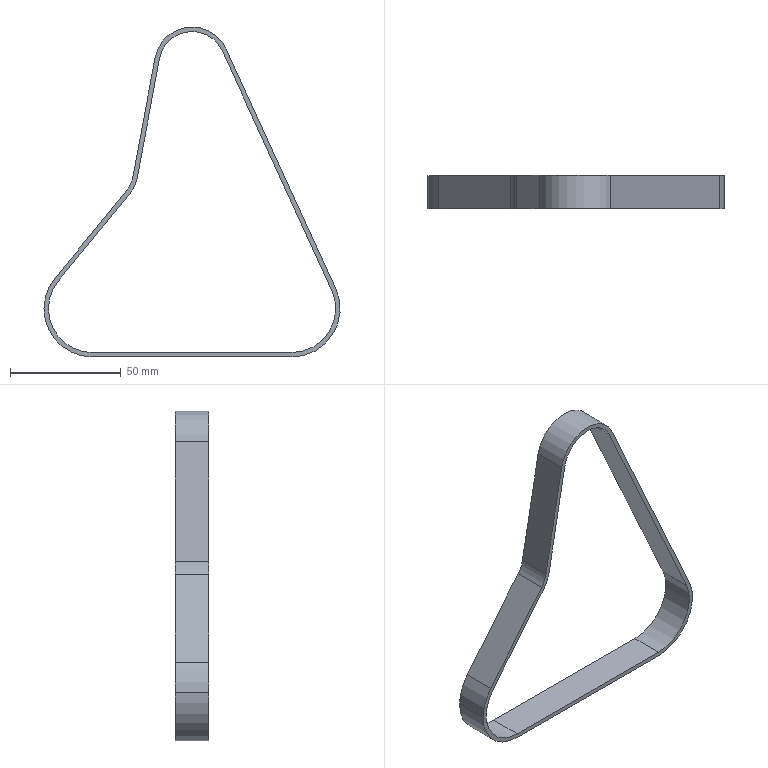Component | SolidWorks | Belt11-1 | 1 solid | 20 faces | box 133.44 x 15 x 148.67 mm | volume 13508 mm3 | cylinder 10 | plane 10 | commonest cylinder face diameters 39.44 x3 43.44 x3 33.89 x1 29.89 x1 26 x1 30 x1
STEP:
#1=COLOUR_RGB('',0.7922,0.8196,0.9333);
#2=FILL_AREA_STYLE_COLOUR('',#1);
#3=FILL_AREA_STYLE('',(#2));
#4=SURFACE_STYLE_FILL_AREA(#3);
#5=SURFACE_SIDE_STYLE('',(#4));
#6=SURFACE_STYLE_USAGE(.BOTH.,#5);
#7=PRESENTATION_STYLE_ASSIGNMENT((#6));
#8=CARTESIAN_POINT('',(-0.317,-0.7841,16.584));
#9=VERTEX_POINT('',#8);
#10=CARTESIAN_POINT('',(-0.4928,-0.7841,16.092));
#11=VERTEX_POINT('',#10);
#12=CARTESIAN_POINT('',(0.2836,-0.7841,16.092));
#13=DIRECTION('',(0.,-1.,0.));
#14=DIRECTION('',(1.,0.,0.));
#15=AXIS2_PLACEMENT_3D('',#12,#13,#14);
#16=CIRCLE('',#15,0.7764);
#17=EDGE_CURVE('',#9,#11,#16,.T.);
#18=ORIENTED_EDGE('',*,*,#17,.T.);
#19=CARTESIAN_POINT('',(-0.4928,-0.1935,16.092));
#20=VERTEX_POINT('',#19);
#21=CARTESIAN_POINT('',(-0.4928,-0.7841,16.092));
#22=DIRECTION('',(0.,1.,0.));
#23=VECTOR('',#22,39.37);
#24=LINE('',#21,#23);
#25=EDGE_CURVE('',#11,#20,#24,.T.);
#26=ORIENTED_EDGE('',*,*,#25,.T.);
#27=CARTESIAN_POINT('',(-0.317,-0.1935,16.584));
#28=VERTEX_POINT('',#27);
#29=CARTESIAN_POINT('',(0.2836,-0.1935,16.092));
#30=DIRECTION('',(0.,-1.,0.));
#31=DIRECTION('',(1.,0.,0.));
#32=AXIS2_PLACEMENT_3D('',#29,#30,#31);
#33=CIRCLE('',#32,0.7764);
#34=EDGE_CURVE('',#28,#20,#33,.T.);
#35=ORIENTED_EDGE('',*,*,#34,.F.);
#36=CARTESIAN_POINT('',(-0.317,-0.7841,16.584));
#37=DIRECTION('',(0.,1.,0.));
#38=VECTOR('',#37,39.37);
#39=LINE('',#36,#38);
#40=EDGE_CURVE('',#9,#28,#39,.T.);
#41=ORIENTED_EDGE('',*,*,#40,.F.);
#42=EDGE_LOOP('',(#18,#26,#35,#41));
#43=FACE_OUTER_BOUND('',#42,.T.);
#44=CARTESIAN_POINT('',(0.2836,-0.7841,16.092));
#45=DIRECTION('',(0.,1.,0.));
#46=DIRECTION('',(-1.,0.,0.));
#47=AXIS2_PLACEMENT_3D('',#44,#45,#46);
#48=CYLINDRICAL_SURFACE('',#47,0.7764);
#49=ADVANCED_FACE('',(#43),#48,.F.);
#50=CARTESIAN_POINT('',(-0.5715,-0.7841,16.092));
#51=VERTEX_POINT('',#50);
#52=CARTESIAN_POINT('',(0.2836,-0.7841,15.237));
#53=VERTEX_POINT('',#52);
#54=CARTESIAN_POINT('',(0.2836,-0.7841,16.092));
#55=DIRECTION('',(0.,-1.,0.));
#56=DIRECTION('',(1.,0.,0.));
#57=AXIS2_PLACEMENT_3D('',#54,#55,#56);
#58=CIRCLE('',#57,0.8551);
#59=EDGE_CURVE('',#51,#53,#58,.T.);
#60=ORIENTED_EDGE('',*,*,#59,.F.);
#61=CARTESIAN_POINT('',(-0.5715,-0.1935,16.092));
#62=VERTEX_POINT('',#61);
#63=CARTESIAN_POINT('',(-0.5715,-0.7841,16.092));
#64=DIRECTION('',(0.,1.,0.));
#65=VECTOR('',#64,39.37);
#66=LINE('',#63,#65);
#67=EDGE_CURVE('',#51,#62,#66,.T.);
#68=ORIENTED_EDGE('',*,*,#67,.T.);
#69=CARTESIAN_POINT('',(0.2836,-0.1935,15.237));
#70=VERTEX_POINT('',#69);
#71=CARTESIAN_POINT('',(0.2836,-0.1935,16.092));
#72=DIRECTION('',(0.,-1.,0.));
#73=DIRECTION('',(1.,0.,0.));
#74=AXIS2_PLACEMENT_3D('',#71,#72,#73);
#75=CIRCLE('',#74,0.8551);
#76=EDGE_CURVE('',#62,#70,#75,.T.);
#77=ORIENTED_EDGE('',*,*,#76,.T.);
#78=CARTESIAN_POINT('',(0.2836,-0.7841,15.237));
#79=DIRECTION('',(0.,1.,0.));
#80=VECTOR('',#79,39.37);
#81=LINE('',#78,#80);
#82=EDGE_CURVE('',#53,#70,#81,.T.);
#83=ORIENTED_EDGE('',*,*,#82,.F.);
#84=EDGE_LOOP('',(#60,#68,#77,#83));
#85=FACE_OUTER_BOUND('',#84,.T.);
#86=CARTESIAN_POINT('',(0.2836,-0.7841,16.092));
#87=DIRECTION('',(0.,1.,0.));
#88=DIRECTION('',(-1.,0.,0.));
#89=AXIS2_PLACEMENT_3D('',#86,#87,#88);
#90=CYLINDRICAL_SURFACE('',#89,0.8551);
#91=ADVANCED_FACE('',(#85),#90,.T.);
#92=ORIENTED_EDGE('',*,*,#17,.F.);
#93=CARTESIAN_POINT('',(0.957,-0.7841,18.139));
#94=VERTEX_POINT('',#93);
#95=CARTESIAN_POINT('',(0.957,-0.7841,18.139));
#96=DIRECTION('',(0.6337,0.,0.7736));
#97=VECTOR('',#96,39.37);
#98=LINE('',#95,#97);
#99=EDGE_CURVE('',#9,#94,#98,.T.);
#100=ORIENTED_EDGE('',*,*,#99,.T.);
#101=CARTESIAN_POINT('',(1.081,-0.7841,18.405));
#102=VERTEX_POINT('',#101);
#103=CARTESIAN_POINT('',(0.5001,-0.7841,18.514));
#104=DIRECTION('',(0.,-1.,0.));
#105=DIRECTION('',(-1.,0.,0.));
#106=AXIS2_PLACEMENT_3D('',#103,#104,#105);
#107=CIRCLE('',#106,0.5906);
#108=EDGE_CURVE('',#94,#102,#107,.T.);
#109=ORIENTED_EDGE('',*,*,#108,.T.);
#110=CARTESIAN_POINT('',(1.477,-0.7841,20.531));
#111=VERTEX_POINT('',#110);
#112=CARTESIAN_POINT('',(1.477,-0.7841,20.531));
#113=DIRECTION('',(0.1832,0.,0.9831));
#114=VECTOR('',#113,39.37);
#115=LINE('',#112,#114);
#116=EDGE_CURVE('',#102,#111,#115,.T.);
#117=ORIENTED_EDGE('',*,*,#116,.T.);
#118=CARTESIAN_POINT('',(2.59,-0.7841,20.668));
#119=VERTEX_POINT('',#118);
#120=CARTESIAN_POINT('',(2.055,-0.7841,20.423));
#121=DIRECTION('',(0.,-1.,0.));
#122=DIRECTION('',(1.,0.,0.));
#123=AXIS2_PLACEMENT_3D('',#120,#121,#122);
#124=CIRCLE('',#123,0.5884);
#125=EDGE_CURVE('',#119,#111,#124,.T.);
#126=ORIENTED_EDGE('',*,*,#125,.F.);
#127=CARTESIAN_POINT('',(4.533,-0.7841,16.415));
#128=VERTEX_POINT('',#127);
#129=CARTESIAN_POINT('',(4.533,-0.7841,16.415));
#130=DIRECTION('',(-0.4155,0.,0.9096));
#131=VECTOR('',#130,39.37);
#132=LINE('',#129,#131);
#133=EDGE_CURVE('',#128,#119,#132,.T.);
#134=ORIENTED_EDGE('',*,*,#133,.F.);
#135=CARTESIAN_POINT('',(3.827,-0.7841,15.316));
#136=VERTEX_POINT('',#135);
#137=CARTESIAN_POINT('',(3.827,-0.7841,16.092));
#138=DIRECTION('',(0.,-1.,0.));
#139=DIRECTION('',(1.,0.,0.));
#140=AXIS2_PLACEMENT_3D('',#137,#138,#139);
#141=CIRCLE('',#140,0.7764);
#142=EDGE_CURVE('',#136,#128,#141,.T.);
#143=ORIENTED_EDGE('',*,*,#142,.F.);
#144=CARTESIAN_POINT('',(0.2836,-0.7841,15.316));
#145=VERTEX_POINT('',#144);
#146=CARTESIAN_POINT('',(0.2836,-0.7841,15.316));
#147=DIRECTION('',(1.,0.,-0.));
#148=VECTOR('',#147,39.37);
#149=LINE('',#146,#148);
#150=EDGE_CURVE('',#145,#136,#149,.T.);
#151=ORIENTED_EDGE('',*,*,#150,.F.);
#152=CARTESIAN_POINT('',(0.2836,-0.7841,16.092));
#153=DIRECTION('',(0.,-1.,0.));
#154=DIRECTION('',(1.,0.,0.));
#155=AXIS2_PLACEMENT_3D('',#152,#153,#154);
#156=CIRCLE('',#155,0.7764);
#157=EDGE_CURVE('',#11,#145,#156,.T.);
#158=ORIENTED_EDGE('',*,*,#157,.F.);
#159=EDGE_LOOP('',(#92,#100,#109,#117,#126,#134,#143,#151,#158));
#160=FACE_BOUND('',#159,.T.);
#161=CARTESIAN_POINT('',(0.896,-0.7841,18.189));
#162=VERTEX_POINT('',#161);
#163=CARTESIAN_POINT('',(-0.3779,-0.7841,16.634));
#164=VERTEX_POINT('',#163);
#165=CARTESIAN_POINT('',(-0.3779,-0.7841,16.634));
#166=DIRECTION('',(-0.6337,0.,-0.7736));
#167=VECTOR('',#166,39.37);
#168=LINE('',#165,#167);
#169=EDGE_CURVE('',#162,#164,#168,.T.);
#170=ORIENTED_EDGE('',*,*,#169,.T.);
#171=CARTESIAN_POINT('',(0.2836,-0.7841,16.092));
#172=DIRECTION('',(0.,-1.,0.));
#173=DIRECTION('',(1.,0.,0.));
#174=AXIS2_PLACEMENT_3D('',#171,#172,#173);
#175=CIRCLE('',#174,0.8551);
#176=EDGE_CURVE('',#164,#51,#175,.T.);
#177=ORIENTED_EDGE('',*,*,#176,.T.);
#178=ORIENTED_EDGE('',*,*,#59,.T.);
#179=CARTESIAN_POINT('',(3.827,-0.7841,15.237));
#180=VERTEX_POINT('',#179);
#181=CARTESIAN_POINT('',(0.2836,-0.7841,15.237));
#182=DIRECTION('',(1.,0.,-0.));
#183=VECTOR('',#182,39.37);
#184=LINE('',#181,#183);
#185=EDGE_CURVE('',#53,#180,#184,.T.);
#186=ORIENTED_EDGE('',*,*,#185,.T.);
#187=CARTESIAN_POINT('',(4.605,-0.7841,16.448));
#188=VERTEX_POINT('',#187);
#189=CARTESIAN_POINT('',(3.827,-0.7841,16.092));
#190=DIRECTION('',(0.,-1.,0.));
#191=DIRECTION('',(1.,0.,0.));
#192=AXIS2_PLACEMENT_3D('',#189,#190,#191);
#193=CIRCLE('',#192,0.8551);
#194=EDGE_CURVE('',#180,#188,#193,.T.);
#195=ORIENTED_EDGE('',*,*,#194,.T.);
#196=CARTESIAN_POINT('',(2.662,-0.7841,20.7));
#197=VERTEX_POINT('',#196);
#198=CARTESIAN_POINT('',(4.605,-0.7841,16.448));
#199=DIRECTION('',(-0.4155,0.,0.9096));
#200=VECTOR('',#199,39.37);
#201=LINE('',#198,#200);
#202=EDGE_CURVE('',#188,#197,#201,.T.);
#203=ORIENTED_EDGE('',*,*,#202,.T.);
#204=CARTESIAN_POINT('',(1.399,-0.7841,20.545));
#205=VERTEX_POINT('',#204);
#206=CARTESIAN_POINT('',(2.055,-0.7841,20.423));
#207=DIRECTION('',(0.,-1.,0.));
#208=DIRECTION('',(1.,0.,0.));
#209=AXIS2_PLACEMENT_3D('',#206,#207,#208);
#210=CIRCLE('',#209,0.6671);
#211=EDGE_CURVE('',#197,#205,#210,.T.);
#212=ORIENTED_EDGE('',*,*,#211,.T.);
#213=CARTESIAN_POINT('',(1.003,-0.7841,18.42));
#214=VERTEX_POINT('',#213);
#215=CARTESIAN_POINT('',(1.003,-0.7841,18.42));
#216=DIRECTION('',(-0.1832,0.,-0.9831));
#217=VECTOR('',#216,39.37);
#218=LINE('',#215,#217);
#219=EDGE_CURVE('',#205,#214,#218,.T.);
#220=ORIENTED_EDGE('',*,*,#219,.T.);
#221=CARTESIAN_POINT('',(0.5001,-0.7841,18.514));
#222=DIRECTION('',(0.,1.,0.));
#223=DIRECTION('',(1.,0.,0.));
#224=AXIS2_PLACEMENT_3D('',#221,#222,#223);
#225=CIRCLE('',#224,0.5118);
#226=EDGE_CURVE('',#214,#162,#225,.T.);
#227=ORIENTED_EDGE('',*,*,#226,.T.);
#228=EDGE_LOOP('',(#170,#177,#178,#186,#195,#203,#212,#220,#227));
#229=FACE_OUTER_BOUND('',#228,.T.);
#230=CARTESIAN_POINT('',(2.055,-0.7841,20.423));
#231=DIRECTION('',(0.,-1.,0.));
#232=DIRECTION('',(1.,0.,0.));
#233=AXIS2_PLACEMENT_3D('',#230,#231,#232);
#234=PLANE('',#233);
#235=ADVANCED_FACE('',(#160,#229),#234,.T.);
#236=CARTESIAN_POINT('',(0.957,-0.1935,18.139));
#237=VERTEX_POINT('',#236);
#238=CARTESIAN_POINT('',(0.957,-0.1935,18.139));
#239=DIRECTION('',(0.6337,0.,0.7736));
#240=VECTOR('',#239,39.37);
#241=LINE('',#238,#240);
#242=EDGE_CURVE('',#28,#237,#241,.T.);
#243=ORIENTED_EDGE('',*,*,#242,.F.);
#244=ORIENTED_EDGE('',*,*,#34,.T.);
#245=CARTESIAN_POINT('',(0.2836,-0.1935,15.316));
#246=VERTEX_POINT('',#245);
#247=CARTESIAN_POINT('',(0.2836,-0.1935,16.092));
#248=DIRECTION('',(0.,-1.,0.));
#249=DIRECTION('',(1.,0.,0.));
#250=AXIS2_PLACEMENT_3D('',#247,#248,#249);
#251=CIRCLE('',#250,0.7764);
#252=EDGE_CURVE('',#20,#246,#251,.T.);
#253=ORIENTED_EDGE('',*,*,#252,.T.);
#254=CARTESIAN_POINT('',(3.827,-0.1935,15.316));
#255=VERTEX_POINT('',#254);
#256=CARTESIAN_POINT('',(0.2836,-0.1935,15.316));
#257=DIRECTION('',(1.,0.,-0.));
#258=VECTOR('',#257,39.37);
#259=LINE('',#256,#258);
#260=EDGE_CURVE('',#246,#255,#259,.T.);
#261=ORIENTED_EDGE('',*,*,#260,.T.);
#262=CARTESIAN_POINT('',(4.533,-0.1935,16.415));
#263=VERTEX_POINT('',#262);
#264=CARTESIAN_POINT('',(3.827,-0.1935,16.092));
#265=DIRECTION('',(0.,-1.,0.));
#266=DIRECTION('',(1.,0.,0.));
#267=AXIS2_PLACEMENT_3D('',#264,#265,#266);
#268=CIRCLE('',#267,0.7764);
#269=EDGE_CURVE('',#255,#263,#268,.T.);
#270=ORIENTED_EDGE('',*,*,#269,.T.);
#271=CARTESIAN_POINT('',(2.59,-0.1935,20.668));
#272=VERTEX_POINT('',#271);
#273=CARTESIAN_POINT('',(4.533,-0.1935,16.415));
#274=DIRECTION('',(-0.4155,0.,0.9096));
#275=VECTOR('',#274,39.37);
#276=LINE('',#273,#275);
#277=EDGE_CURVE('',#263,#272,#276,.T.);
#278=ORIENTED_EDGE('',*,*,#277,.T.);
#279=CARTESIAN_POINT('',(1.477,-0.1935,20.531));
#280=VERTEX_POINT('',#279);
#281=CARTESIAN_POINT('',(2.055,-0.1935,20.423));
#282=DIRECTION('',(0.,-1.,0.));
#283=DIRECTION('',(1.,0.,0.));
#284=AXIS2_PLACEMENT_3D('',#281,#282,#283);
#285=CIRCLE('',#284,0.5884);
#286=EDGE_CURVE('',#272,#280,#285,.T.);
#287=ORIENTED_EDGE('',*,*,#286,.T.);
#288=CARTESIAN_POINT('',(1.081,-0.1935,18.405));
#289=VERTEX_POINT('',#288);
#290=CARTESIAN_POINT('',(1.477,-0.1935,20.531));
#291=DIRECTION('',(0.1832,0.,0.9831));
#292=VECTOR('',#291,39.37);
#293=LINE('',#290,#292);
#294=EDGE_CURVE('',#289,#280,#293,.T.);
#295=ORIENTED_EDGE('',*,*,#294,.F.);
#296=CARTESIAN_POINT('',(0.5001,-0.1935,18.514));
#297=DIRECTION('',(0.,-1.,0.));
#298=DIRECTION('',(-1.,0.,0.));
#299=AXIS2_PLACEMENT_3D('',#296,#297,#298);
#300=CIRCLE('',#299,0.5906);
#301=EDGE_CURVE('',#237,#289,#300,.T.);
#302=ORIENTED_EDGE('',*,*,#301,.F.);
#303=EDGE_LOOP('',(#243,#244,#253,#261,#270,#278,#287,#295,#302));
#304=FACE_BOUND('',#303,.T.);
#305=CARTESIAN_POINT('',(-0.3779,-0.1935,16.634));
#306=VERTEX_POINT('',#305);
#307=CARTESIAN_POINT('',(0.2836,-0.1935,16.092));
#308=DIRECTION('',(0.,-1.,0.));
#309=DIRECTION('',(1.,0.,0.));
#310=AXIS2_PLACEMENT_3D('',#307,#308,#309);
#311=CIRCLE('',#310,0.8551);
#312=EDGE_CURVE('',#306,#62,#311,.T.);
#313=ORIENTED_EDGE('',*,*,#312,.F.);
#314=CARTESIAN_POINT('',(0.896,-0.1935,18.189));
#315=VERTEX_POINT('',#314);
#316=CARTESIAN_POINT('',(-0.3779,-0.1935,16.634));
#317=DIRECTION('',(-0.6337,0.,-0.7736));
#318=VECTOR('',#317,39.37);
#319=LINE('',#316,#318);
#320=EDGE_CURVE('',#315,#306,#319,.T.);
#321=ORIENTED_EDGE('',*,*,#320,.F.);
#322=CARTESIAN_POINT('',(1.003,-0.1935,18.42));
#323=VERTEX_POINT('',#322);
#324=CARTESIAN_POINT('',(0.5001,-0.1935,18.514));
#325=DIRECTION('',(0.,1.,0.));
#326=DIRECTION('',(1.,0.,0.));
#327=AXIS2_PLACEMENT_3D('',#324,#325,#326);
#328=CIRCLE('',#327,0.5118);
#329=EDGE_CURVE('',#323,#315,#328,.T.);
#330=ORIENTED_EDGE('',*,*,#329,.F.);
#331=CARTESIAN_POINT('',(1.399,-0.1935,20.545));
#332=VERTEX_POINT('',#331);
#333=CARTESIAN_POINT('',(1.003,-0.1935,18.42));
#334=DIRECTION('',(-0.1832,0.,-0.9831));
#335=VECTOR('',#334,39.37);
#336=LINE('',#333,#335);
#337=EDGE_CURVE('',#332,#323,#336,.T.);
#338=ORIENTED_EDGE('',*,*,#337,.F.);
#339=CARTESIAN_POINT('',(2.662,-0.1935,20.7));
#340=VERTEX_POINT('',#339);
#341=CARTESIAN_POINT('',(2.055,-0.1935,20.423));
#342=DIRECTION('',(0.,-1.,0.));
#343=DIRECTION('',(1.,0.,0.));
#344=AXIS2_PLACEMENT_3D('',#341,#342,#343);
#345=CIRCLE('',#344,0.6671);
#346=EDGE_CURVE('',#340,#332,#345,.T.);
#347=ORIENTED_EDGE('',*,*,#346,.F.);
#348=CARTESIAN_POINT('',(4.605,-0.1935,16.448));
#349=VERTEX_POINT('',#348);
#350=CARTESIAN_POINT('',(4.605,-0.1935,16.448));
#351=DIRECTION('',(-0.4155,0.,0.9096));
#352=VECTOR('',#351,39.37);
#353=LINE('',#350,#352);
#354=EDGE_CURVE('',#349,#340,#353,.T.);
#355=ORIENTED_EDGE('',*,*,#354,.F.);
#356=CARTESIAN_POINT('',(3.827,-0.1935,15.237));
#357=VERTEX_POINT('',#356);
#358=CARTESIAN_POINT('',(3.827,-0.1935,16.092));
#359=DIRECTION('',(0.,-1.,0.));
#360=DIRECTION('',(1.,0.,0.));
#361=AXIS2_PLACEMENT_3D('',#358,#359,#360);
#362=CIRCLE('',#361,0.8551);
#363=EDGE_CURVE('',#357,#349,#362,.T.);
#364=ORIENTED_EDGE('',*,*,#363,.F.);
#365=CARTESIAN_POINT('',(0.2836,-0.1935,15.237));
#366=DIRECTION('',(1.,0.,-0.));
#367=VECTOR('',#366,39.37);
#368=LINE('',#365,#367);
#369=EDGE_CURVE('',#70,#357,#368,.T.);
#370=ORIENTED_EDGE('',*,*,#369,.F.);
#371=ORIENTED_EDGE('',*,*,#76,.F.);
#372=EDGE_LOOP('',(#313,#321,#330,#338,#347,#355,#364,#370,#371));
#373=FACE_OUTER_BOUND('',#372,.T.);
#374=CARTESIAN_POINT('',(2.055,-0.1935,20.423));
#375=DIRECTION('',(0.,-1.,0.));
#376=DIRECTION('',(1.,0.,0.));
#377=AXIS2_PLACEMENT_3D('',#374,#375,#376);
#378=PLANE('',#377);
#379=ADVANCED_FACE('',(#304,#373),#378,.F.);
#380=ORIENTED_EDGE('',*,*,#346,.T.);
#381=CARTESIAN_POINT('',(1.399,-0.7841,20.545));
#382=DIRECTION('',(0.,1.,0.));
#383=VECTOR('',#382,39.37);
#384=LINE('',#381,#383);
#385=EDGE_CURVE('',#205,#332,#384,.T.);
#386=ORIENTED_EDGE('',*,*,#385,.F.);
#387=ORIENTED_EDGE('',*,*,#211,.F.);
#388=CARTESIAN_POINT('',(2.662,-0.7841,20.7));
#389=DIRECTION('',(0.,1.,0.));
#390=VECTOR('',#389,39.37);
#391=LINE('',#388,#390);
#392=EDGE_CURVE('',#197,#340,#391,.T.);
#393=ORIENTED_EDGE('',*,*,#392,.T.);
#394=EDGE_LOOP('',(#380,#386,#387,#393));
#395=FACE_OUTER_BOUND('',#394,.T.);
#396=CARTESIAN_POINT('',(2.055,-0.7841,20.423));
#397=DIRECTION('',(0.,1.,0.));
#398=DIRECTION('',(-1.,0.,0.));
#399=AXIS2_PLACEMENT_3D('',#396,#397,#398);
#400=CYLINDRICAL_SURFACE('',#399,0.6671);
#401=ADVANCED_FACE('',(#395),#400,.T.);
#402=ORIENTED_EDGE('',*,*,#67,.F.);
#403=ORIENTED_EDGE('',*,*,#176,.F.);
#404=CARTESIAN_POINT('',(-0.3779,-0.7841,16.634));
#405=DIRECTION('',(0.,1.,0.));
#406=VECTOR('',#405,39.37);
#407=LINE('',#404,#406);
#408=EDGE_CURVE('',#164,#306,#407,.T.);
#409=ORIENTED_EDGE('',*,*,#408,.T.);
#410=ORIENTED_EDGE('',*,*,#312,.T.);
#411=EDGE_LOOP('',(#402,#403,#409,#410));
#412=FACE_OUTER_BOUND('',#411,.T.);
#413=CARTESIAN_POINT('',(0.2836,-0.7841,16.092));
#414=DIRECTION('',(0.,1.,0.));
#415=DIRECTION('',(-1.,0.,0.));
#416=AXIS2_PLACEMENT_3D('',#413,#414,#415);
#417=CYLINDRICAL_SURFACE('',#416,0.8551);
#418=ADVANCED_FACE('',(#412),#417,.T.);
#419=ORIENTED_EDGE('',*,*,#369,.T.);
#420=CARTESIAN_POINT('',(3.827,-0.7841,15.237));
#421=DIRECTION('',(0.,1.,0.));
#422=VECTOR('',#421,39.37);
#423=LINE('',#420,#422);
#424=EDGE_CURVE('',#180,#357,#423,.T.);
#425=ORIENTED_EDGE('',*,*,#424,.F.);
#426=ORIENTED_EDGE('',*,*,#185,.F.);
#427=ORIENTED_EDGE('',*,*,#82,.T.);
#428=EDGE_LOOP('',(#419,#425,#426,#427));
#429=FACE_OUTER_BOUND('',#428,.T.);
#430=CARTESIAN_POINT('',(0.2836,-0.7841,15.237));
#431=DIRECTION('',(0.,0.,1.));
#432=DIRECTION('',(-1.,0.,0.));
#433=AXIS2_PLACEMENT_3D('',#430,#431,#432);
#434=PLANE('',#433);
#435=ADVANCED_FACE('',(#429),#434,.F.);
#436=ORIENTED_EDGE('',*,*,#363,.T.);
#437=CARTESIAN_POINT('',(4.605,-0.7841,16.448));
#438=DIRECTION('',(0.,1.,0.));
#439=VECTOR('',#438,39.37);
#440=LINE('',#437,#439);
#441=EDGE_CURVE('',#188,#349,#440,.T.);
#442=ORIENTED_EDGE('',*,*,#441,.F.);
#443=ORIENTED_EDGE('',*,*,#194,.F.);
#444=ORIENTED_EDGE('',*,*,#424,.T.);
#445=EDGE_LOOP('',(#436,#442,#443,#444));
#446=FACE_OUTER_BOUND('',#445,.T.);
#447=CARTESIAN_POINT('',(3.827,-0.7841,16.092));
#448=DIRECTION('',(0.,1.,0.));
#449=DIRECTION('',(-1.,0.,0.));
#450=AXIS2_PLACEMENT_3D('',#447,#448,#449);
#451=CYLINDRICAL_SURFACE('',#450,0.8551);
#452=ADVANCED_FACE('',(#446),#451,.T.);
#453=ORIENTED_EDGE('',*,*,#354,.T.);
#454=ORIENTED_EDGE('',*,*,#392,.F.);
#455=ORIENTED_EDGE('',*,*,#202,.F.);
#456=ORIENTED_EDGE('',*,*,#441,.T.);
#457=EDGE_LOOP('',(#453,#454,#455,#456));
#458=FACE_OUTER_BOUND('',#457,.T.);
#459=CARTESIAN_POINT('',(4.605,-0.7841,16.448));
#460=DIRECTION('',(-0.9096,0.,-0.4155));
#461=DIRECTION('',(0.4155,0.,-0.9096));
#462=AXIS2_PLACEMENT_3D('',#459,#460,#461);
#463=PLANE('',#462);
#464=ADVANCED_FACE('',(#458),#463,.F.);
#465=ORIENTED_EDGE('',*,*,#286,.F.);
#466=CARTESIAN_POINT('',(2.59,-0.7841,20.668));
#467=DIRECTION('',(0.,1.,0.));
#468=VECTOR('',#467,39.37);
#469=LINE('',#466,#468);
#470=EDGE_CURVE('',#119,#272,#469,.T.);
#471=ORIENTED_EDGE('',*,*,#470,.F.);
#472=ORIENTED_EDGE('',*,*,#125,.T.);
#473=CARTESIAN_POINT('',(1.477,-0.7841,20.531));
#474=DIRECTION('',(0.,1.,0.));
#475=VECTOR('',#474,39.37);
#476=LINE('',#473,#475);
#477=EDGE_CURVE('',#111,#280,#476,.T.);
#478=ORIENTED_EDGE('',*,*,#477,.T.);
#479=EDGE_LOOP('',(#465,#471,#472,#478));
#480=FACE_OUTER_BOUND('',#479,.T.);
#481=CARTESIAN_POINT('',(2.055,-0.7841,20.423));
#482=DIRECTION('',(0.,1.,0.));
#483=DIRECTION('',(-1.,0.,0.));
#484=AXIS2_PLACEMENT_3D('',#481,#482,#483);
#485=CYLINDRICAL_SURFACE('',#484,0.5884);
#486=ADVANCED_FACE('',(#480),#485,.F.);
#487=ORIENTED_EDGE('',*,*,#25,.F.);
#488=ORIENTED_EDGE('',*,*,#157,.T.);
#489=CARTESIAN_POINT('',(0.2836,-0.7841,15.316));
#490=DIRECTION('',(0.,1.,0.));
#491=VECTOR('',#490,39.37);
#492=LINE('',#489,#491);
#493=EDGE_CURVE('',#145,#246,#492,.T.);
#494=ORIENTED_EDGE('',*,*,#493,.T.);
#495=ORIENTED_EDGE('',*,*,#252,.F.);
#496=EDGE_LOOP('',(#487,#488,#494,#495));
#497=FACE_OUTER_BOUND('',#496,.T.);
#498=CARTESIAN_POINT('',(0.2836,-0.7841,16.092));
#499=DIRECTION('',(0.,1.,0.));
#500=DIRECTION('',(-1.,0.,0.));
#501=AXIS2_PLACEMENT_3D('',#498,#499,#500);
#502=CYLINDRICAL_SURFACE('',#501,0.7764);
#503=ADVANCED_FACE('',(#497),#502,.F.);
#504=ORIENTED_EDGE('',*,*,#260,.F.);
#505=ORIENTED_EDGE('',*,*,#493,.F.);
#506=ORIENTED_EDGE('',*,*,#150,.T.);
#507=CARTESIAN_POINT('',(3.827,-0.7841,15.316));
#508=DIRECTION('',(0.,1.,0.));
#509=VECTOR('',#508,39.37);
#510=LINE('',#507,#509);
#511=EDGE_CURVE('',#136,#255,#510,.T.);
#512=ORIENTED_EDGE('',*,*,#511,.T.);
#513=EDGE_LOOP('',(#504,#505,#506,#512));
#514=FACE_OUTER_BOUND('',#513,.T.);
#515=CARTESIAN_POINT('',(0.2836,-0.7841,15.316));
#516=DIRECTION('',(0.,0.,1.));
#517=DIRECTION('',(-1.,0.,0.));
#518=AXIS2_PLACEMENT_3D('',#515,#516,#517);
#519=PLANE('',#518);
#520=ADVANCED_FACE('',(#514),#519,.T.);
#521=ORIENTED_EDGE('',*,*,#269,.F.);
#522=ORIENTED_EDGE('',*,*,#511,.F.);
#523=ORIENTED_EDGE('',*,*,#142,.T.);
#524=CARTESIAN_POINT('',(4.533,-0.7841,16.415));
#525=DIRECTION('',(0.,1.,0.));
#526=VECTOR('',#525,39.37);
#527=LINE('',#524,#526);
#528=EDGE_CURVE('',#128,#263,#527,.T.);
#529=ORIENTED_EDGE('',*,*,#528,.T.);
#530=EDGE_LOOP('',(#521,#522,#523,#529));
#531=FACE_OUTER_BOUND('',#530,.T.);
#532=CARTESIAN_POINT('',(3.827,-0.7841,16.092));
#533=DIRECTION('',(0.,1.,0.));
#534=DIRECTION('',(-1.,0.,0.));
#535=AXIS2_PLACEMENT_3D('',#532,#533,#534);
#536=CYLINDRICAL_SURFACE('',#535,0.7764);
#537=ADVANCED_FACE('',(#531),#536,.F.);
#538=ORIENTED_EDGE('',*,*,#277,.F.);
#539=ORIENTED_EDGE('',*,*,#528,.F.);
#540=ORIENTED_EDGE('',*,*,#133,.T.);
#541=ORIENTED_EDGE('',*,*,#470,.T.);
#542=EDGE_LOOP('',(#538,#539,#540,#541));
#543=FACE_OUTER_BOUND('',#542,.T.);
#544=CARTESIAN_POINT('',(4.533,-0.7841,16.415));
#545=DIRECTION('',(-0.9096,0.,-0.4155));
#546=DIRECTION('',(0.4155,0.,-0.9096));
#547=AXIS2_PLACEMENT_3D('',#544,#545,#546);
#548=PLANE('',#547);
#549=ADVANCED_FACE('',(#543),#548,.T.);
#550=ORIENTED_EDGE('',*,*,#337,.T.);
#551=CARTESIAN_POINT('',(1.003,-0.7841,18.42));
#552=DIRECTION('',(0.,1.,0.));
#553=VECTOR('',#552,39.37);
#554=LINE('',#551,#553);
#555=EDGE_CURVE('',#214,#323,#554,.T.);
#556=ORIENTED_EDGE('',*,*,#555,.F.);
#557=ORIENTED_EDGE('',*,*,#219,.F.);
#558=ORIENTED_EDGE('',*,*,#385,.T.);
#559=EDGE_LOOP('',(#550,#556,#557,#558));
#560=FACE_OUTER_BOUND('',#559,.T.);
#561=CARTESIAN_POINT('',(1.003,-0.7841,18.42));
#562=DIRECTION('',(0.9831,0.,-0.1832));
#563=DIRECTION('',(0.1832,0.,0.9831));
#564=AXIS2_PLACEMENT_3D('',#561,#562,#563);
#565=PLANE('',#564);
#566=ADVANCED_FACE('',(#560),#565,.F.);
#567=ORIENTED_EDGE('',*,*,#329,.T.);
#568=CARTESIAN_POINT('',(0.896,-0.7841,18.189));
#569=DIRECTION('',(0.,1.,0.));
#570=VECTOR('',#569,39.37);
#571=LINE('',#568,#570);
#572=EDGE_CURVE('',#162,#315,#571,.T.);
#573=ORIENTED_EDGE('',*,*,#572,.F.);
#574=ORIENTED_EDGE('',*,*,#226,.F.);
#575=ORIENTED_EDGE('',*,*,#555,.T.);
#576=EDGE_LOOP('',(#567,#573,#574,#575));
#577=FACE_OUTER_BOUND('',#576,.T.);
#578=CARTESIAN_POINT('',(0.5001,-0.7841,18.514));
#579=DIRECTION('',(0.,1.,0.));
#580=DIRECTION('',(-1.,0.,0.));
#581=AXIS2_PLACEMENT_3D('',#578,#579,#580);
#582=CYLINDRICAL_SURFACE('',#581,0.5118);
#583=ADVANCED_FACE('',(#577),#582,.F.);
#584=ORIENTED_EDGE('',*,*,#320,.T.);
#585=ORIENTED_EDGE('',*,*,#408,.F.);
#586=ORIENTED_EDGE('',*,*,#169,.F.);
#587=ORIENTED_EDGE('',*,*,#572,.T.);
#588=EDGE_LOOP('',(#584,#585,#586,#587));
#589=FACE_OUTER_BOUND('',#588,.T.);
#590=CARTESIAN_POINT('',(-0.3779,-0.7841,16.634));
#591=DIRECTION('',(0.7736,0.,-0.6337));
#592=DIRECTION('',(0.6337,0.,0.7736));
#593=AXIS2_PLACEMENT_3D('',#590,#591,#592);
#594=PLANE('',#593);
#595=ADVANCED_FACE('',(#589),#594,.F.);
#596=ORIENTED_EDGE('',*,*,#242,.T.);
#597=CARTESIAN_POINT('',(0.957,-0.7841,18.139));
#598=DIRECTION('',(0.,1.,0.));
#599=VECTOR('',#598,39.37);
#600=LINE('',#597,#599);
#601=EDGE_CURVE('',#94,#237,#600,.T.);
#602=ORIENTED_EDGE('',*,*,#601,.F.);
#603=ORIENTED_EDGE('',*,*,#99,.F.);
#604=ORIENTED_EDGE('',*,*,#40,.T.);
#605=EDGE_LOOP('',(#596,#602,#603,#604));
#606=FACE_OUTER_BOUND('',#605,.T.);
#607=CARTESIAN_POINT('',(0.957,-0.7841,18.139));
#608=DIRECTION('',(-0.7736,0.,0.6337));
#609=DIRECTION('',(-0.6337,0.,-0.7736));
#610=AXIS2_PLACEMENT_3D('',#607,#608,#609);
#611=PLANE('',#610);
#612=ADVANCED_FACE('',(#606),#611,.F.);
#613=ORIENTED_EDGE('',*,*,#301,.T.);
#614=CARTESIAN_POINT('',(1.081,-0.7841,18.405));
#615=DIRECTION('',(0.,1.,0.));
#616=VECTOR('',#615,39.37);
#617=LINE('',#614,#616);
#618=EDGE_CURVE('',#102,#289,#617,.T.);
#619=ORIENTED_EDGE('',*,*,#618,.F.);
#620=ORIENTED_EDGE('',*,*,#108,.F.);
#621=ORIENTED_EDGE('',*,*,#601,.T.);
#622=EDGE_LOOP('',(#613,#619,#620,#621));
#623=FACE_OUTER_BOUND('',#622,.T.);
#624=CARTESIAN_POINT('',(0.5001,-0.7841,18.514));
#625=DIRECTION('',(0.,1.,0.));
#626=DIRECTION('',(-1.,0.,0.));
#627=AXIS2_PLACEMENT_3D('',#624,#625,#626);
#628=CYLINDRICAL_SURFACE('',#627,0.5906);
#629=ADVANCED_FACE('',(#623),#628,.T.);
#630=ORIENTED_EDGE('',*,*,#294,.T.);
#631=ORIENTED_EDGE('',*,*,#477,.F.);
#632=ORIENTED_EDGE('',*,*,#116,.F.);
#633=ORIENTED_EDGE('',*,*,#618,.T.);
#634=EDGE_LOOP('',(#630,#631,#632,#633));
#635=FACE_OUTER_BOUND('',#634,.T.);
#636=CARTESIAN_POINT('',(1.477,-0.7841,20.531));
#637=DIRECTION('',(-0.9831,0.,0.1832));
#638=DIRECTION('',(-0.1832,0.,-0.9831));
#639=AXIS2_PLACEMENT_3D('',#636,#637,#638);
#640=PLANE('',#639);
#641=ADVANCED_FACE('',(#635),#640,.F.);
#642=CLOSED_SHELL('',(#49,#91,#235,#379,#401,#418,#435,#452,#464,#486,#503,#520,#537,#549,#566,#583,#595,#612,#629,#641));
#643=MANIFOLD_SOLID_BREP('',#642);
#644=STYLED_ITEM('',(#7),#643);
#645=PRESENTATION_LAYER_ASSIGNMENT('','',(#644));
#646=(LENGTH_UNIT()NAMED_UNIT(*)SI_UNIT($,.METRE.));
#647=LENGTH_MEASURE_WITH_UNIT(LENGTH_MEASURE(0.0254),#646);
#648=DIMENSIONAL_EXPONENTS(1.,0.,0.,0.,0.,0.,0.);
#649=(CONVERSION_BASED_UNIT('',#647)LENGTH_UNIT()NAMED_UNIT(#648));
#650=UNCERTAINTY_MEASURE_WITH_UNIT(LENGTH_MEASURE(0.00001),#649,'','');
#651=(NAMED_UNIT(*)PLANE_ANGLE_UNIT()SI_UNIT($,.RADIAN.));
#652=(NAMED_UNIT(*)SI_UNIT($,.STERADIAN.)SOLID_ANGLE_UNIT());
#653=(GEOMETRIC_REPRESENTATION_CONTEXT(3)GLOBAL_UNCERTAINTY_ASSIGNED_CONTEXT((#650))GLOBAL_UNIT_ASSIGNED_CONTEXT((#649,#651,#652))REPRESENTATION_CONTEXT('',''));
#654=MECHANICAL_DESIGN_GEOMETRIC_PRESENTATION_REPRESENTATION('',(#644),#653);
#655=CARTESIAN_POINT('',(0.,0.,0.));
#656=DIRECTION('',(0.,0.,1.));
#657=DIRECTION('',(1.,0.,0.));
#658=AXIS2_PLACEMENT_3D('',#655,#656,#657);
#659=(LENGTH_UNIT()NAMED_UNIT(*)SI_UNIT($,.METRE.));
#660=LENGTH_MEASURE_WITH_UNIT(LENGTH_MEASURE(0.0254),#659);
#661=DIMENSIONAL_EXPONENTS(1.,0.,0.,0.,0.,0.,0.);
#662=(CONVERSION_BASED_UNIT('',#660)LENGTH_UNIT()NAMED_UNIT(#661));
#663=UNCERTAINTY_MEASURE_WITH_UNIT(LENGTH_MEASURE(0.00001),#662,'','');
#664=(NAMED_UNIT(*)PLANE_ANGLE_UNIT()SI_UNIT($,.RADIAN.));
#665=(NAMED_UNIT(*)SI_UNIT($,.STERADIAN.)SOLID_ANGLE_UNIT());
#666=(GEOMETRIC_REPRESENTATION_CONTEXT(3)GLOBAL_UNCERTAINTY_ASSIGNED_CONTEXT((#663))GLOBAL_UNIT_ASSIGNED_CONTEXT((#662,#664,#665))REPRESENTATION_CONTEXT('',''));
#667=ADVANCED_BREP_SHAPE_REPRESENTATION('',(#643,#658),#666);